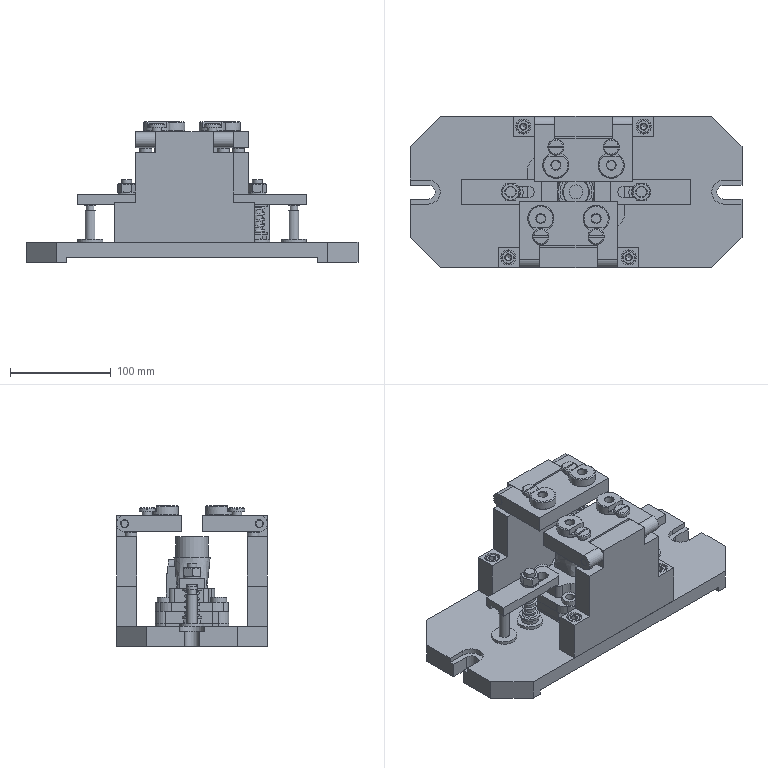Assembly | NX | mm | 53 component files | 53 solids | 867 faces | box 330 x 150 x 140 mm | volume 1574748 mm3 | plane 420 | cylinder 223 | cone 198 | spline 12 | torus 12 | sphere 2 | commonest cylinder face diameters 8 x30 20 x25 10 x20 6 x19 9 x14 15 x14 16 x12 11 x10
Bill of materials:
GB-T6173-2000,M10x1 | 2 |  | Low-profile hexagonal prism with a central through-bore; both end faces have chamfered corners, giving the shape of a thin hex nut.
unnamed part 1 | 2 |  | Plain solid cylindrical rod with flat ends; long and slender.
GB-T70.1-2000,M8x40 | 4 |  | Hexagon Socket Head Cap Screw, GB-T 70.1-2000,M8x40
unnamed part 2 | 4 |  | Solid stepped round part: a large chamfered disc-like head, a short narrower neck, and a smaller cylindrical body that is chamfered at its free end.
unnamed part 3 | 2 |  | Flat rectangular bar with a through obround slot near one end. That end has chamfered corners, and there is a shallow stepped recess on the underside near the slotted end.
GB-T95-2002,M10 | 4 |  | Plain Washer, GB-T 95-2002,M10
unnamed part 4 | 4 |  | Slotted-head stepped pin: a wide round head with a straight slot across it, a cylindrical shoulder below the head, a narrow neck, and a smaller chamfered cylindrical tip.
GB-T6170_F-2000,M10x1.5 | 2 |  | Hexagonal nut-like body with a central round through bore and chamfered corners on both faces.
unnamed part 5 | 1 |  | Flanged housing: a lobed base flange with mounting holes, a raised rectangular pad, a tapered tubular boss with a counterbored central bore, and a small side lug with a hole.
unnamed part 6 | 1 |  | Flat plate with a rectangular central area and two diagonally opposite rounded ears. The central area has four holes, and each ear has a counterbored hole.
unnamed part 7 | 1 |  | Solid stepped pin: a round chamfered head, a neck, a thin wide integral flange or collar, another neck, and a chamfered cylindrical lower section.
unnamed part 8 | 4 |  | Plain cylindrical sleeve (tube) with a through bore and small chamfers on the outer and inner edges at both ends.
GB-T70.1-2000,M8x12 | 2 |  | Hexagon Socket Head Cap Screw, GB-T 70.1-2000,M8x12
unnamed part 9 | 1 |  | Flat elongated plate with chamfered corners (octagon-like outline) and an open U-slot at each short end. It has several counterbored holes along the centerline, small through holes near the long edges, a thin groove or step line, and an obround recess on the top face.
unnamed part 10 | 1 |  | Solid stepped pin with a hexagonal head: a chamfered hex section on top, a neck, a thin wide integral flange, another neck, and a chamfered cylindrical lower section.
unnamed part 11 | 2 |  | Helical coil spring of round wire with a constant coil diameter and roughly six active coils. The ends appear closed and flattened.
GB-T848-2002,M10 | 2 |  | Thin flat annular disc (ring) with a concentric circular through-hole and plain cylindrical edges, matching a plain flat washer shape.
unnamed part 12 | 4 |  | Flanged cylindrical bushing-like part: a wide round head with chamfered edges sits on a smaller cylindrical shank. A coaxial through-bore runs through it, and a flat cut on one side of the head forms a step.
unnamed part 13 | 2 |  | Rectangular plate-like block with a rectangular notch cut into one edge, which leaves two prongs. Each prong ends in a rounded, knuckle-like end with a cross hole along the prong-end axis. The main body has two large through-holes and two small countersunk holes.
GB-T119.1-2000,8x22 | 2 |  | Parallel Pin, GB-T 119.1-2000,8x22
unnamed part 14 | 2 |  | Long, narrow prismatic block with a stepped, symmetric profile shaped like a pyramid, built from three levels: a full-length base, a shorter middle tier and a shortest top tier. The base ends and the middle-tier shoulders carry vertical holes, and the top tier has a transverse hole near one end.
GB-T119.1-2000,8x80 | 2 |  | Parallel Pin, GB-T 119.1-2000,8x80
unnamed part 15 | 2 |  | Cylindrical pin with a domed, slightly larger round head. Under the head is a short neck that is smaller in diameter than the shank, forming a groove. Below the neck is a long plain cylindrical shank with a flat end.
Mates:
1. fix | jig_body 1 component
2. concentric | datum_block 1 edge | jig_body 1 edge
3. touch align | A_stud 2 face | clamp_plate 2 face
4. touch align | clamp_plate 2 face | control_cover 1 face
5. center | clamp_plate 2 face | clamp_plate 2 face | control_cover 1 face | control_cover 1 face
6. touch align | control_cover 1 face | datum_block 1 face
7. touch align | datum_block 1 face | jig_body 1 face
8. distance | clamp_plate 2 face | control_cover 1 face
9. distance | A_stud 2 face | clamp_plate 2 face
10. touch align | B_stud 2 face | jig_body 1 face
11. touch align | B_stud 2 face | clamp_plate 2 face
12. concentric | GB-T95-2002_M10 4 edge | GB-T6173-2000_M10x1 2 edge
13. concentric | GB-T6173-2000_M10x1 2 edge | jig_body 1 edge
14. concentric | GB-T848-2002_M10 2 edge | clamp_plate 2 edge
15. concentric | GB-T6170_F-2000_M10x1_5 2 edge | GB-T848-2002_M10 2 edge
16. touch align | GB-T95-2002_M10 3 face | A_stud 2 face
17. touch align | GB-T95-2002_M10 3 face | clamp_plate 2 face
18. concentric | spring 2 edge | GB-T95-2002_M10 4 edge
19. bond | control_cover 1 component | assembly component
20. bond | clamp_plate 2 component | assembly component
21. bond | B_stud 2 component | assembly component
22. bond | GB-T95-2002_M10 4 component | assembly component
23. bond | GB-T848-2002_M10 2 component | assembly component
24. bond | GB-T6170_F-2000_M10x1_5 2 component | assembly component
25. bond | GB-T6173-2000_M10x1 2 component | assembly component
26. bond | clamp_plate 1 component | assembly component
27. bond | B_stud 1 component | assembly component
28. bond | GB-T95-2002_M10 2 component | assembly component
29. bond | GB-T848-2002_M10 1 component | assembly component
30. bond | GB-T6170_F-2000_M10x1_5 1 component | assembly component
31. bond | GB-T6173-2000_M10x1 1 component | assembly component
32. circular | assembly datumaxis | assembly cartesiancoordinatesystem | assembly cartesiancoordinatesystem
33. circular | assembly datumaxis | assembly cartesiancoordinatesystem | assembly cartesiancoordinatesystem
34. circular | assembly datumaxis | assembly cartesiancoordinatesystem | assembly cartesiancoordinatesystem
35. circular | assembly datumaxis | assembly cartesiancoordinatesystem | assembly cartesiancoordinatesystem
36. circular | assembly datumaxis | assembly cartesiancoordinatesystem | assembly cartesiancoordinatesystem
37. circular | assembly datumaxis | assembly cartesiancoordinatesystem | assembly cartesiancoordinatesystem
38. bond | A_stud 2 component | assembly component
39. bond | A_stud 1 component | assembly component
40. circular | assembly datumaxis | assembly cartesiancoordinatesystem | assembly cartesiancoordinatesystem
41. bond | GB-T95-2002_M10 3 component | assembly component
42. bond | GB-T95-2002_M10 1 component | assembly component
43. circular | assembly datumaxis | assembly cartesiancoordinatesystem | assembly cartesiancoordinatesystem
44. concentric | spring 1 edge | GB-T95-2002_M10 2 edge
45. concentric | diamond_pin 1 edge | datum_block 1 edge
46. concentric | dowel_pin 1 edge | datum_block 1 edge
47. concentric | bushing 4 edge | drill_bushing 4 edge
48. concentric | drill_bushing 4 edge | drill_template 2 edge
49. touch align | drill_bushing 4 face | control_cover 1 face
50. bond | drill_template 2 component | assembly component
51. bond | drill_bushing 4 component | assembly component
52. bond | bushing 4 component | assembly component
53. bond | drill_bushing 3 component | assembly component
54. bond | bushing 3 component | assembly component
55. linear | assembly datumaxis | assembly cartesiancoordinatesystem | assembly cartesiancoordinatesystem
56. linear | assembly datumaxis | assembly cartesiancoordinatesystem | assembly cartesiancoordinatesystem
57. touch align | bracket 2 face | jig_body 1 face
58. center | bracket 2 face | bracket 2 face | drill_template 2 face | drill_template 2 face
59. touch align | drill_template 2 face | bracket 2 face
60. touch align | bracket 2 face | jig_body 1 face
61. concentric | support_pin 4 edge | bracket 2 edge
62. concentric | support_pin 3 edge | bracket 2 edge
63. concentric | drill_bushing_screw 4 edge | drill_template 2 arc
64. bond | drill_bushing_screw 4 component | assembly component
65. bond | drill_bushing_screw 3 component | assembly component
66. linear | assembly datumaxis | assembly cartesiancoordinatesystem | assembly cartesiancoordinatesystem
67. bond | drill_bushing_screw 4 component | assembly component
68. bond | drill_bushing_screw 2 component | assembly component
69. circular | assembly datumaxis | assembly cartesiancoordinatesystem | assembly cartesiancoordinatesystem
70. bond | drill_bushing 4 component | assembly component
71. bond | drill_bushing 2 component | assembly component
72. circular | assembly datumaxis | assembly cartesiancoordinatesystem | assembly cartesiancoordinatesystem
73. bond | drill_bushing 3 component | assembly component
74. bond | drill_bushing 1 component | assembly component
75. circular | assembly datumaxis | assembly cartesiancoordinatesystem | assembly cartesiancoordinatesystem
76. bond | drill_bushing_screw 3 component | assembly component
77. bond | drill_bushing_screw 1 component | assembly component
78. circular | assembly datumaxis | assembly cartesiancoordinatesystem | assembly cartesiancoordinatesystem
79. bond | drill_template 2 component | assembly component
80. bond | drill_template 1 component | assembly component
81. circular | assembly datumaxis | assembly cartesiancoordinatesystem | assembly cartesiancoordinatesystem
82. bond | bracket 2 component | assembly component
83. bond | bracket 1 component | assembly component
84. circular | assembly datumaxis | assembly cartesiancoordinatesystem | assembly cartesiancoordinatesystem
85. bond | bushing 4 component | assembly component
86. bond | bushing 2 component | assembly component
87. circular | assembly datumaxis | assembly cartesiancoordinatesystem | assembly cartesiancoordinatesystem
88. bond | bushing 3 component | assembly component
89. bond | bushing 1 component | assembly component
90. circular | assembly datumaxis | assembly cartesiancoordinatesystem | assembly cartesiancoordinatesystem
91. bond | support_pin 4 component | assembly component
92. bond | support_pin 2 component | assembly component
93. circular | assembly datumaxis | assembly cartesiancoordinatesystem | assembly cartesiancoordinatesystem
94. bond | support_pin 3 component | assembly component
95. bond | support_pin 1 component | assembly component
96. circular | assembly datumaxis | assembly cartesiancoordinatesystem | assembly cartesiancoordinatesystem
97. bond | hinge 2 component | assembly component
98. bond | hinge 1 component | assembly component
99. circular | assembly datumaxis | assembly cartesiancoordinatesystem | assembly cartesiancoordinatesystem
100. bond | GB-T70_1-2000_M8x40 4 component | assembly component
101. bond | GB-T70_1-2000_M8x40 2 component | assembly component
102. circular | assembly datumaxis | assembly cartesiancoordinatesystem | assembly cartesiancoordinatesystem
103. bond | GB-T70_1-2000_M8x40 3 component | assembly component
104. bond | GB-T70_1-2000_M8x40 1 component | assembly component
105. circular | assembly datumaxis | assembly cartesiancoordinatesystem | assembly cartesiancoordinatesystem